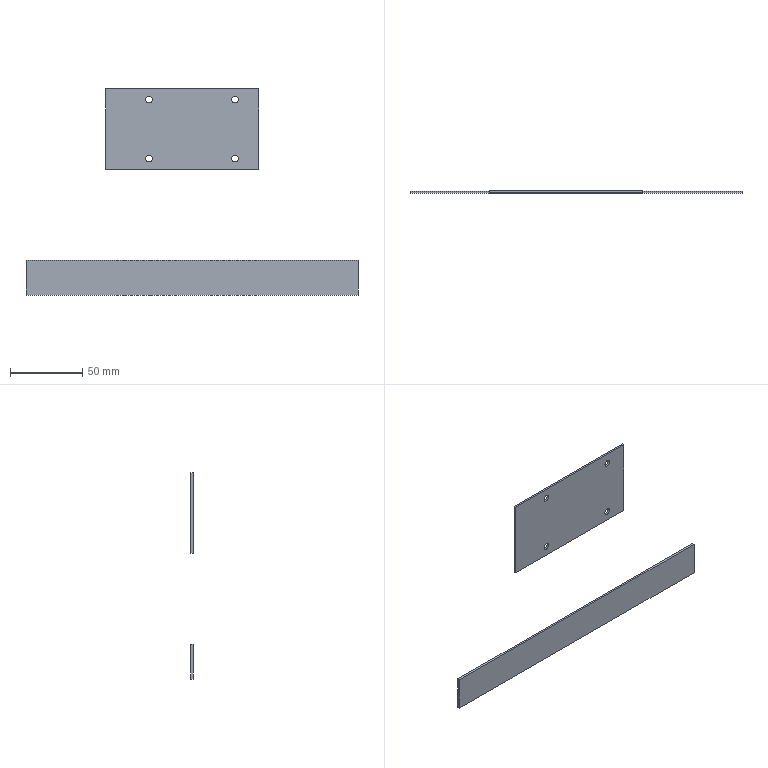Component | SolidWorks | CopperGasket-1 | 2 solids | 20 faces | box 230 x 1.5 x 142.89 mm | volume 17087 mm3 | plane 12 | cylinder 8 | commonest cylinder face diameters 4.542 x8
build123d program:
from build123d import *

# Parameters (mm, degrees)
SKETCH1_W           = 24.104
SKETCH1_H           = 230
BOSS_EXTRUDE1_DEPTH = 1.5
SKETCH3_W           = 55.775
SKETCH3_H           = 106
BOSS_EXTRUDE2_DEPTH = 1.5
SKETCH2_R           = 2.271
CUT_EXTRUDE1_DEPTH  = 210.219


with BuildPart() as part:
    # Sketch1 → Boss-Extrude1 (new body)
    with BuildSketch(Plane.XY):
        with Locations((102.948, -59.772)):
            Rectangle(SKETCH1_W, SKETCH1_H)
    extrude(amount=BOSS_EXTRUDE1_DEPTH)


with BuildPart() as body_2:
    # Sketch3 → Boss-Extrude2 (new body)
    with BuildSketch(Plane.XY.offset(1.5)):
        with Locations((0, -53)):
            Rectangle(SKETCH3_W, SKETCH3_H)
    extrude(amount=-BOSS_EXTRUDE2_DEPTH)

    # Sketch2 → Cut-Extrude1 (cut, through all)
    with BuildSketch(Plane.XY.offset(1.5)):
        with Locations((20.473, -29.973)):
            Circle(SKETCH2_R)
        with Locations((20.473, -89.571)):
            Circle(SKETCH2_R)
        with Locations((-20.473, -29.973)):
            Circle(SKETCH2_R)
        with Locations((-20.473, -89.571)):
            Circle(SKETCH2_R)
    extrude(amount=-CUT_EXTRUDE1_DEPTH, mode=Mode.SUBTRACT)


solid = Compound([part.part, body_2.part])

# Placed as in the assembly
solid = solid.moved(Location((-3, 95.24, 0), (-90, 0, 90)))
STEP:
#1=COLOUR_RGB('',0.7922,0.8196,0.9333);
#2=FILL_AREA_STYLE_COLOUR('',#1);
#3=FILL_AREA_STYLE('',(#2));
#4=SURFACE_STYLE_FILL_AREA(#3);
#5=SURFACE_SIDE_STYLE('',(#4));
#6=SURFACE_STYLE_USAGE(.BOTH.,#5);
#7=PRESENTATION_STYLE_ASSIGNMENT((#6));
#8=CARTESIAN_POINT('',(-2.292,3.75,-4.528));
#9=VERTEX_POINT('',#8);
#10=CARTESIAN_POINT('',(-2.292,3.75,-3.579));
#11=VERTEX_POINT('',#10);
#12=CARTESIAN_POINT('',(-2.292,3.75,-4.528));
#13=DIRECTION('',(0.,-0.,1.));
#14=VECTOR('',#13,39.37);
#15=LINE('',#12,#14);
#16=EDGE_CURVE('',#9,#11,#15,.T.);
#17=ORIENTED_EDGE('',*,*,#16,.T.);
#18=CARTESIAN_POINT('',(-2.292,3.809,-3.579));
#19=VERTEX_POINT('',#18);
#20=CARTESIAN_POINT('',(-2.292,3.809,-3.579));
#21=DIRECTION('',(0.,-1.,-0.));
#22=VECTOR('',#21,39.37);
#23=LINE('',#20,#22);
#24=EDGE_CURVE('',#19,#11,#23,.T.);
#25=ORIENTED_EDGE('',*,*,#24,.F.);
#26=CARTESIAN_POINT('',(-2.292,3.809,-4.528));
#27=VERTEX_POINT('',#26);
#28=CARTESIAN_POINT('',(-2.292,3.809,-4.528));
#29=DIRECTION('',(0.,-0.,1.));
#30=VECTOR('',#29,39.37);
#31=LINE('',#28,#30);
#32=EDGE_CURVE('',#27,#19,#31,.T.);
#33=ORIENTED_EDGE('',*,*,#32,.F.);
#34=CARTESIAN_POINT('',(-2.292,3.809,-4.528));
#35=DIRECTION('',(0.,-1.,-0.));
#36=VECTOR('',#35,39.37);
#37=LINE('',#34,#36);
#38=EDGE_CURVE('',#27,#9,#37,.T.);
#39=ORIENTED_EDGE('',*,*,#38,.T.);
#40=EDGE_LOOP('',(#17,#25,#33,#39));
#41=FACE_OUTER_BOUND('',#40,.T.);
#42=CARTESIAN_POINT('',(-2.292,3.809,-4.528));
#43=DIRECTION('',(1.,0.,-0.));
#44=DIRECTION('',(0.,-1.,-0.));
#45=AXIS2_PLACEMENT_3D('',#42,#43,#44);
#46=PLANE('',#45);
#47=ADVANCED_FACE('',(#41),#46,.F.);
#48=CARTESIAN_POINT('',(6.763,3.75,-3.579));
#49=VERTEX_POINT('',#48);
#50=CARTESIAN_POINT('',(-2.292,3.75,-3.579));
#51=DIRECTION('',(1.,-0.,0.));
#52=VECTOR('',#51,39.37);
#53=LINE('',#50,#52);
#54=EDGE_CURVE('',#11,#49,#53,.T.);
#55=ORIENTED_EDGE('',*,*,#54,.T.);
#56=CARTESIAN_POINT('',(6.763,3.809,-3.579));
#57=VERTEX_POINT('',#56);
#58=CARTESIAN_POINT('',(6.763,3.809,-3.579));
#59=DIRECTION('',(0.,-1.,-0.));
#60=VECTOR('',#59,39.37);
#61=LINE('',#58,#60);
#62=EDGE_CURVE('',#57,#49,#61,.T.);
#63=ORIENTED_EDGE('',*,*,#62,.F.);
#64=CARTESIAN_POINT('',(-2.292,3.809,-3.579));
#65=DIRECTION('',(1.,-0.,0.));
#66=VECTOR('',#65,39.37);
#67=LINE('',#64,#66);
#68=EDGE_CURVE('',#19,#57,#67,.T.);
#69=ORIENTED_EDGE('',*,*,#68,.F.);
#70=ORIENTED_EDGE('',*,*,#24,.T.);
#71=EDGE_LOOP('',(#55,#63,#69,#70));
#72=FACE_OUTER_BOUND('',#71,.T.);
#73=CARTESIAN_POINT('',(-2.292,3.809,-3.579));
#74=DIRECTION('',(0.,0.,-1.));
#75=DIRECTION('',(-1.,0.,-0.));
#76=AXIS2_PLACEMENT_3D('',#73,#74,#75);
#77=PLANE('',#76);
#78=ADVANCED_FACE('',(#72),#77,.F.);
#79=CARTESIAN_POINT('',(6.763,3.75,-4.528));
#80=VERTEX_POINT('',#79);
#81=CARTESIAN_POINT('',(6.763,3.75,-3.579));
#82=DIRECTION('',(0.,0.,-1.));
#83=VECTOR('',#82,39.37);
#84=LINE('',#81,#83);
#85=EDGE_CURVE('',#49,#80,#84,.T.);
#86=ORIENTED_EDGE('',*,*,#85,.T.);
#87=CARTESIAN_POINT('',(6.763,3.809,-4.528));
#88=VERTEX_POINT('',#87);
#89=CARTESIAN_POINT('',(6.763,3.809,-4.528));
#90=DIRECTION('',(0.,-1.,-0.));
#91=VECTOR('',#90,39.37);
#92=LINE('',#89,#91);
#93=EDGE_CURVE('',#88,#80,#92,.T.);
#94=ORIENTED_EDGE('',*,*,#93,.F.);
#95=CARTESIAN_POINT('',(6.763,3.809,-3.579));
#96=DIRECTION('',(0.,0.,-1.));
#97=VECTOR('',#96,39.37);
#98=LINE('',#95,#97);
#99=EDGE_CURVE('',#57,#88,#98,.T.);
#100=ORIENTED_EDGE('',*,*,#99,.F.);
#101=ORIENTED_EDGE('',*,*,#62,.T.);
#102=EDGE_LOOP('',(#86,#94,#100,#101));
#103=FACE_OUTER_BOUND('',#102,.T.);
#104=CARTESIAN_POINT('',(6.763,3.809,-3.579));
#105=DIRECTION('',(-1.,-0.,0.));
#106=DIRECTION('',(0.,1.,0.));
#107=AXIS2_PLACEMENT_3D('',#104,#105,#106);
#108=PLANE('',#107);
#109=ADVANCED_FACE('',(#103),#108,.F.);
#110=CARTESIAN_POINT('',(6.763,3.75,-4.528));
#111=DIRECTION('',(-1.,-0.,0.));
#112=VECTOR('',#111,39.37);
#113=LINE('',#110,#112);
#114=EDGE_CURVE('',#80,#9,#113,.T.);
#115=ORIENTED_EDGE('',*,*,#114,.T.);
#116=ORIENTED_EDGE('',*,*,#38,.F.);
#117=CARTESIAN_POINT('',(6.763,3.809,-4.528));
#118=DIRECTION('',(-1.,-0.,0.));
#119=VECTOR('',#118,39.37);
#120=LINE('',#117,#119);
#121=EDGE_CURVE('',#88,#27,#120,.T.);
#122=ORIENTED_EDGE('',*,*,#121,.F.);
#123=ORIENTED_EDGE('',*,*,#93,.T.);
#124=EDGE_LOOP('',(#115,#116,#122,#123));
#125=FACE_OUTER_BOUND('',#124,.T.);
#126=CARTESIAN_POINT('',(6.763,3.809,-4.528));
#127=DIRECTION('',(0.,-0.,1.));
#128=DIRECTION('',(1.,0.,-0.));
#129=AXIS2_PLACEMENT_3D('',#126,#127,#128);
#130=PLANE('',#129);
#131=ADVANCED_FACE('',(#125),#130,.F.);
#132=ORIENTED_EDGE('',*,*,#32,.T.);
#133=ORIENTED_EDGE('',*,*,#68,.T.);
#134=ORIENTED_EDGE('',*,*,#99,.T.);
#135=ORIENTED_EDGE('',*,*,#121,.T.);
#136=EDGE_LOOP('',(#132,#133,#134,#135));
#137=FACE_OUTER_BOUND('',#136,.T.);
#138=CARTESIAN_POINT('',(-0.1181,3.809,0.));
#139=DIRECTION('',(0.,1.,0.));
#140=DIRECTION('',(0.,0.,-1.));
#141=AXIS2_PLACEMENT_3D('',#138,#139,#140);
#142=PLANE('',#141);
#143=ADVANCED_FACE('',(#137),#142,.T.);
#144=ORIENTED_EDGE('',*,*,#16,.F.);
#145=ORIENTED_EDGE('',*,*,#114,.F.);
#146=ORIENTED_EDGE('',*,*,#85,.F.);
#147=ORIENTED_EDGE('',*,*,#54,.F.);
#148=EDGE_LOOP('',(#144,#145,#146,#147));
#149=FACE_OUTER_BOUND('',#148,.T.);
#150=CARTESIAN_POINT('',(-0.1181,3.75,0.));
#151=DIRECTION('',(0.,1.,0.));
#152=DIRECTION('',(0.,0.,-1.));
#153=AXIS2_PLACEMENT_3D('',#150,#151,#152);
#154=PLANE('',#153);
#155=ADVANCED_FACE('',(#149),#154,.F.);
#156=CLOSED_SHELL('',(#47,#78,#109,#131,#143,#155));
#157=MANIFOLD_SOLID_BREP('',#156);
#158=STYLED_ITEM('',(#7),#157);
#159=PRESENTATION_LAYER_ASSIGNMENT('','',(#158));
#160=(LENGTH_UNIT()NAMED_UNIT(*)SI_UNIT($,.METRE.));
#161=LENGTH_MEASURE_WITH_UNIT(LENGTH_MEASURE(0.0254),#160);
#162=DIMENSIONAL_EXPONENTS(1.,0.,0.,0.,0.,0.,0.);
#163=(CONVERSION_BASED_UNIT('',#161)LENGTH_UNIT()NAMED_UNIT(#162));
#164=UNCERTAINTY_MEASURE_WITH_UNIT(LENGTH_MEASURE(0.00001),#163,'','');
#165=(NAMED_UNIT(*)PLANE_ANGLE_UNIT()SI_UNIT($,.RADIAN.));
#166=(NAMED_UNIT(*)SI_UNIT($,.STERADIAN.)SOLID_ANGLE_UNIT());
#167=(GEOMETRIC_REPRESENTATION_CONTEXT(3)GLOBAL_UNCERTAINTY_ASSIGNED_CONTEXT((#164))GLOBAL_UNIT_ASSIGNED_CONTEXT((#163,#165,#166))REPRESENTATION_CONTEXT('',''));
#168=MECHANICAL_DESIGN_GEOMETRIC_PRESENTATION_REPRESENTATION('',(#158),#167);
#169=COLOUR_RGB('',0.7922,0.8196,0.9333);
#170=FILL_AREA_STYLE_COLOUR('',#169);
#171=FILL_AREA_STYLE('',(#170));
#172=SURFACE_STYLE_FILL_AREA(#171);
#173=SURFACE_SIDE_STYLE('',(#172));
#174=SURFACE_STYLE_USAGE(.BOTH.,#173);
#175=PRESENTATION_STYLE_ASSIGNMENT((#174));
#176=CARTESIAN_POINT('',(3.408,3.75,-0.7166));
#177=VERTEX_POINT('',#176);
#178=CARTESIAN_POINT('',(3.408,3.75,-0.8954));
#179=VERTEX_POINT('',#178);
#180=CARTESIAN_POINT('',(3.408,3.75,-0.806));
#181=DIRECTION('',(0.,1.,0.));
#182=DIRECTION('',(0.,0.,-1.));
#183=AXIS2_PLACEMENT_3D('',#180,#181,#182);
#184=CIRCLE('',#183,0.08941);
#185=EDGE_CURVE('',#177,#179,#184,.T.);
#186=ORIENTED_EDGE('',*,*,#185,.F.);
#187=CARTESIAN_POINT('',(3.408,3.809,-0.7166));
#188=VERTEX_POINT('',#187);
#189=CARTESIAN_POINT('',(3.408,3.75,-0.7166));
#190=DIRECTION('',(0.,1.,0.));
#191=VECTOR('',#190,39.37);
#192=LINE('',#189,#191);
#193=EDGE_CURVE('',#177,#188,#192,.T.);
#194=ORIENTED_EDGE('',*,*,#193,.T.);
#195=CARTESIAN_POINT('',(3.408,3.809,-0.8954));
#196=VERTEX_POINT('',#195);
#197=CARTESIAN_POINT('',(3.408,3.809,-0.806));
#198=DIRECTION('',(0.,1.,0.));
#199=DIRECTION('',(0.,0.,-1.));
#200=AXIS2_PLACEMENT_3D('',#197,#198,#199);
#201=CIRCLE('',#200,0.08941);
#202=EDGE_CURVE('',#188,#196,#201,.T.);
#203=ORIENTED_EDGE('',*,*,#202,.T.);
#204=CARTESIAN_POINT('',(3.408,3.75,-0.8954));
#205=DIRECTION('',(0.,1.,0.));
#206=VECTOR('',#205,39.37);
#207=LINE('',#204,#206);
#208=EDGE_CURVE('',#179,#196,#207,.T.);
#209=ORIENTED_EDGE('',*,*,#208,.F.);
#210=EDGE_LOOP('',(#186,#194,#203,#209));
#211=FACE_OUTER_BOUND('',#210,.T.);
#212=CARTESIAN_POINT('',(3.408,3.75,-0.806));
#213=DIRECTION('',(0.,1.,0.));
#214=DIRECTION('',(0.,0.,-1.));
#215=AXIS2_PLACEMENT_3D('',#212,#213,#214);
#216=CYLINDRICAL_SURFACE('',#215,0.08941);
#217=ADVANCED_FACE('',(#211),#216,.F.);
#218=CARTESIAN_POINT('',(1.062,3.75,0.8954));
#219=VERTEX_POINT('',#218);
#220=CARTESIAN_POINT('',(1.062,3.75,0.7166));
#221=VERTEX_POINT('',#220);
#222=CARTESIAN_POINT('',(1.062,3.75,0.806));
#223=DIRECTION('',(0.,1.,0.));
#224=DIRECTION('',(0.,0.,-1.));
#225=AXIS2_PLACEMENT_3D('',#222,#223,#224);
#226=CIRCLE('',#225,0.08941);
#227=EDGE_CURVE('',#219,#221,#226,.T.);
#228=ORIENTED_EDGE('',*,*,#227,.F.);
#229=CARTESIAN_POINT('',(1.062,3.809,0.8954));
#230=VERTEX_POINT('',#229);
#231=CARTESIAN_POINT('',(1.062,3.75,0.8954));
#232=DIRECTION('',(0.,1.,0.));
#233=VECTOR('',#232,39.37);
#234=LINE('',#231,#233);
#235=EDGE_CURVE('',#219,#230,#234,.T.);
#236=ORIENTED_EDGE('',*,*,#235,.T.);
#237=CARTESIAN_POINT('',(1.062,3.809,0.7166));
#238=VERTEX_POINT('',#237);
#239=CARTESIAN_POINT('',(1.062,3.809,0.806));
#240=DIRECTION('',(0.,1.,0.));
#241=DIRECTION('',(0.,0.,-1.));
#242=AXIS2_PLACEMENT_3D('',#239,#240,#241);
#243=CIRCLE('',#242,0.08941);
#244=EDGE_CURVE('',#230,#238,#243,.T.);
#245=ORIENTED_EDGE('',*,*,#244,.T.);
#246=CARTESIAN_POINT('',(1.062,3.75,0.7166));
#247=DIRECTION('',(0.,1.,0.));
#248=VECTOR('',#247,39.37);
#249=LINE('',#246,#248);
#250=EDGE_CURVE('',#221,#238,#249,.T.);
#251=ORIENTED_EDGE('',*,*,#250,.F.);
#252=EDGE_LOOP('',(#228,#236,#245,#251));
#253=FACE_OUTER_BOUND('',#252,.T.);
#254=CARTESIAN_POINT('',(1.062,3.75,0.806));
#255=DIRECTION('',(0.,1.,0.));
#256=DIRECTION('',(0.,0.,-1.));
#257=AXIS2_PLACEMENT_3D('',#254,#255,#256);
#258=CYLINDRICAL_SURFACE('',#257,0.08941);
#259=ADVANCED_FACE('',(#253),#258,.F.);
#260=CARTESIAN_POINT('',(3.408,3.75,0.8954));
#261=VERTEX_POINT('',#260);
#262=CARTESIAN_POINT('',(3.408,3.75,0.7166));
#263=VERTEX_POINT('',#262);
#264=CARTESIAN_POINT('',(3.408,3.75,0.806));
#265=DIRECTION('',(0.,1.,0.));
#266=DIRECTION('',(0.,0.,-1.));
#267=AXIS2_PLACEMENT_3D('',#264,#265,#266);
#268=CIRCLE('',#267,0.08941);
#269=EDGE_CURVE('',#261,#263,#268,.T.);
#270=ORIENTED_EDGE('',*,*,#269,.F.);
#271=CARTESIAN_POINT('',(3.408,3.809,0.8954));
#272=VERTEX_POINT('',#271);
#273=CARTESIAN_POINT('',(3.408,3.75,0.8954));
#274=DIRECTION('',(0.,1.,0.));
#275=VECTOR('',#274,39.37);
#276=LINE('',#273,#275);
#277=EDGE_CURVE('',#261,#272,#276,.T.);
#278=ORIENTED_EDGE('',*,*,#277,.T.);
#279=CARTESIAN_POINT('',(3.408,3.809,0.7166));
#280=VERTEX_POINT('',#279);
#281=CARTESIAN_POINT('',(3.408,3.809,0.806));
#282=DIRECTION('',(0.,1.,0.));
#283=DIRECTION('',(0.,0.,-1.));
#284=AXIS2_PLACEMENT_3D('',#281,#282,#283);
#285=CIRCLE('',#284,0.08941);
#286=EDGE_CURVE('',#272,#280,#285,.T.);
#287=ORIENTED_EDGE('',*,*,#286,.T.);
#288=CARTESIAN_POINT('',(3.408,3.75,0.7166));
#289=DIRECTION('',(0.,1.,0.));
#290=VECTOR('',#289,39.37);
#291=LINE('',#288,#290);
#292=EDGE_CURVE('',#263,#280,#291,.T.);
#293=ORIENTED_EDGE('',*,*,#292,.F.);
#294=EDGE_LOOP('',(#270,#278,#287,#293));
#295=FACE_OUTER_BOUND('',#294,.T.);
#296=CARTESIAN_POINT('',(3.408,3.75,0.806));
#297=DIRECTION('',(0.,1.,0.));
#298=DIRECTION('',(0.,0.,-1.));
#299=AXIS2_PLACEMENT_3D('',#296,#297,#298);
#300=CYLINDRICAL_SURFACE('',#299,0.08941);
#301=ADVANCED_FACE('',(#295),#300,.F.);
#302=CARTESIAN_POINT('',(1.062,3.75,-0.7166));
#303=VERTEX_POINT('',#302);
#304=CARTESIAN_POINT('',(1.062,3.75,-0.8954));
#305=VERTEX_POINT('',#304);
#306=CARTESIAN_POINT('',(1.062,3.75,-0.806));
#307=DIRECTION('',(0.,1.,0.));
#308=DIRECTION('',(0.,0.,-1.));
#309=AXIS2_PLACEMENT_3D('',#306,#307,#308);
#310=CIRCLE('',#309,0.08941);
#311=EDGE_CURVE('',#303,#305,#310,.T.);
#312=ORIENTED_EDGE('',*,*,#311,.F.);
#313=CARTESIAN_POINT('',(1.062,3.809,-0.7166));
#314=VERTEX_POINT('',#313);
#315=CARTESIAN_POINT('',(1.062,3.75,-0.7166));
#316=DIRECTION('',(0.,1.,0.));
#317=VECTOR('',#316,39.37);
#318=LINE('',#315,#317);
#319=EDGE_CURVE('',#303,#314,#318,.T.);
#320=ORIENTED_EDGE('',*,*,#319,.T.);
#321=CARTESIAN_POINT('',(1.062,3.809,-0.8954));
#322=VERTEX_POINT('',#321);
#323=CARTESIAN_POINT('',(1.062,3.809,-0.806));
#324=DIRECTION('',(0.,1.,0.));
#325=DIRECTION('',(0.,0.,-1.));
#326=AXIS2_PLACEMENT_3D('',#323,#324,#325);
#327=CIRCLE('',#326,0.08941);
#328=EDGE_CURVE('',#314,#322,#327,.T.);
#329=ORIENTED_EDGE('',*,*,#328,.T.);
#330=CARTESIAN_POINT('',(1.062,3.75,-0.8954));
#331=DIRECTION('',(0.,1.,0.));
#332=VECTOR('',#331,39.37);
#333=LINE('',#330,#332);
#334=EDGE_CURVE('',#305,#322,#333,.T.);
#335=ORIENTED_EDGE('',*,*,#334,.F.);
#336=EDGE_LOOP('',(#312,#320,#329,#335));
#337=FACE_OUTER_BOUND('',#336,.T.);
#338=CARTESIAN_POINT('',(1.062,3.75,-0.806));
#339=DIRECTION('',(0.,1.,0.));
#340=DIRECTION('',(0.,0.,-1.));
#341=AXIS2_PLACEMENT_3D('',#338,#339,#340);
#342=CYLINDRICAL_SURFACE('',#341,0.08941);
#343=ADVANCED_FACE('',(#337),#342,.F.);
#344=CARTESIAN_POINT('',(4.055,3.809,1.098));
#345=VERTEX_POINT('',#344);
#346=CARTESIAN_POINT('',(-0.1181,3.809,1.098));
#347=VERTEX_POINT('',#346);
#348=CARTESIAN_POINT('',(-0.1181,3.809,1.098));
#349=DIRECTION('',(-1.,0.,0.));
#350=VECTOR('',#349,39.37);
#351=LINE('',#348,#350);
#352=EDGE_CURVE('',#345,#347,#351,.T.);
#353=ORIENTED_EDGE('',*,*,#352,.T.);
#354=CARTESIAN_POINT('',(-0.1181,3.75,1.098));
#355=VERTEX_POINT('',#354);
#356=CARTESIAN_POINT('',(-0.1181,3.75,1.098));
#357=DIRECTION('',(0.,1.,0.));
#358=VECTOR('',#357,39.37);
#359=LINE('',#356,#358);
#360=EDGE_CURVE('',#355,#347,#359,.T.);
#361=ORIENTED_EDGE('',*,*,#360,.F.);
#362=CARTESIAN_POINT('',(4.055,3.75,1.098));
#363=VERTEX_POINT('',#362);
#364=CARTESIAN_POINT('',(-0.1181,3.75,1.098));
#365=DIRECTION('',(-1.,0.,0.));
#366=VECTOR('',#365,39.37);
#367=LINE('',#364,#366);
#368=EDGE_CURVE('',#363,#355,#367,.T.);
#369=ORIENTED_EDGE('',*,*,#368,.F.);
#370=CARTESIAN_POINT('',(4.055,3.75,1.098));
#371=DIRECTION('',(0.,1.,0.));
#372=VECTOR('',#371,39.37);
#373=LINE('',#370,#372);
#374=EDGE_CURVE('',#363,#345,#373,.T.);
#375=ORIENTED_EDGE('',*,*,#374,.T.);
#376=EDGE_LOOP('',(#353,#361,#369,#375));
#377=FACE_OUTER_BOUND('',#376,.T.);
#378=CARTESIAN_POINT('',(-0.1181,3.75,1.098));
#379=DIRECTION('',(0.,0.,-1.));
#380=DIRECTION('',(0.,-1.,-0.));
#381=AXIS2_PLACEMENT_3D('',#378,#379,#380);
#382=PLANE('',#381);
#383=ADVANCED_FACE('',(#377),#382,.F.);
#384=CARTESIAN_POINT('',(-0.1181,3.809,-1.098));
#385=VERTEX_POINT('',#384);
#386=CARTESIAN_POINT('',(-0.1181,3.809,0.));
#387=DIRECTION('',(0.,-0.,1.));
#388=VECTOR('',#387,39.37);
#389=LINE('',#386,#388);
#390=EDGE_CURVE('',#385,#347,#389,.T.);
#391=ORIENTED_EDGE('',*,*,#390,.F.);
#392=CARTESIAN_POINT('',(-0.1181,3.75,-1.098));
#393=VERTEX_POINT('',#392);
#394=CARTESIAN_POINT('',(-0.1181,3.75,-1.098));
#395=DIRECTION('',(0.,1.,0.));
#396=VECTOR('',#395,39.37);
#397=LINE('',#394,#396);
#398=EDGE_CURVE('',#393,#385,#397,.T.);
#399=ORIENTED_EDGE('',*,*,#398,.F.);
#400=CARTESIAN_POINT('',(-0.1181,3.75,0.));
#401=DIRECTION('',(0.,-0.,1.));
#402=VECTOR('',#401,39.37);
#403=LINE('',#400,#402);
#404=EDGE_CURVE('',#393,#355,#403,.T.);
#405=ORIENTED_EDGE('',*,*,#404,.T.);
#406=ORIENTED_EDGE('',*,*,#360,.T.);
#407=EDGE_LOOP('',(#391,#399,#405,#406));
#408=FACE_OUTER_BOUND('',#407,.T.);
#409=CARTESIAN_POINT('',(-0.1181,3.75,0.));
#410=DIRECTION('',(-1.,-0.,0.));
#411=DIRECTION('',(0.,1.,0.));
#412=AXIS2_PLACEMENT_3D('',#409,#410,#411);
#413=PLANE('',#412);
#414=ADVANCED_FACE('',(#408),#413,.T.);
#415=CARTESIAN_POINT('',(4.055,3.809,-1.098));
#416=VERTEX_POINT('',#415);
#417=CARTESIAN_POINT('',(-0.1181,3.809,-1.098));
#418=DIRECTION('',(-1.,0.,0.));
#419=VECTOR('',#418,39.37);
#420=LINE('',#417,#419);
#421=EDGE_CURVE('',#416,#385,#420,.T.);
#422=ORIENTED_EDGE('',*,*,#421,.F.);
#423=CARTESIAN_POINT('',(4.055,3.75,-1.098));
#424=VERTEX_POINT('',#423);
#425=CARTESIAN_POINT('',(4.055,3.75,-1.098));
#426=DIRECTION('',(0.,1.,0.));
#427=VECTOR('',#426,39.37);
#428=LINE('',#425,#427);
#429=EDGE_CURVE('',#424,#416,#428,.T.);
#430=ORIENTED_EDGE('',*,*,#429,.F.);
#431=CARTESIAN_POINT('',(-0.1181,3.75,-1.098));
#432=DIRECTION('',(-1.,0.,0.));
#433=VECTOR('',#432,39.37);
#434=LINE('',#431,#433);
#435=EDGE_CURVE('',#424,#393,#434,.T.);
#436=ORIENTED_EDGE('',*,*,#435,.T.);
#437=ORIENTED_EDGE('',*,*,#398,.T.);
#438=EDGE_LOOP('',(#422,#430,#436,#437));
#439=FACE_OUTER_BOUND('',#438,.T.);
#440=CARTESIAN_POINT('',(-0.1181,3.75,-1.098));
#441=DIRECTION('',(0.,0.,-1.));
#442=DIRECTION('',(0.,-1.,-0.));
#443=AXIS2_PLACEMENT_3D('',#440,#441,#442);
#444=PLANE('',#443);
#445=ADVANCED_FACE('',(#439),#444,.T.);
#446=CARTESIAN_POINT('',(4.055,3.809,0.));
#447=DIRECTION('',(0.,-0.,1.));
#448=VECTOR('',#447,39.37);
#449=LINE('',#446,#448);
#450=EDGE_CURVE('',#416,#345,#449,.T.);
#451=ORIENTED_EDGE('',*,*,#450,.T.);
#452=ORIENTED_EDGE('',*,*,#374,.F.);
#453=CARTESIAN_POINT('',(4.055,3.75,0.));
#454=DIRECTION('',(0.,-0.,1.));
#455=VECTOR('',#454,39.37);
#456=LINE('',#453,#455);
#457=EDGE_CURVE('',#424,#363,#456,.T.);
#458=ORIENTED_EDGE('',*,*,#457,.F.);
#459=ORIENTED_EDGE('',*,*,#429,.T.);
#460=EDGE_LOOP('',(#451,#452,#458,#459));
#461=FACE_OUTER_BOUND('',#460,.T.);
#462=CARTESIAN_POINT('',(4.055,3.75,0.));
#463=DIRECTION('',(-1.,-0.,0.));
#464=DIRECTION('',(0.,1.,0.));
#465=AXIS2_PLACEMENT_3D('',#462,#463,#464);
#466=PLANE('',#465);
#467=ADVANCED_FACE('',(#461),#466,.F.);
#468=CARTESIAN_POINT('',(3.408,3.75,-0.806));
#469=DIRECTION('',(0.,1.,0.));
#470=DIRECTION('',(0.,0.,-1.));
#471=AXIS2_PLACEMENT_3D('',#468,#469,#470);
#472=CIRCLE('',#471,0.08941);
#473=EDGE_CURVE('',#179,#177,#472,.T.);
#474=ORIENTED_EDGE('',*,*,#473,.T.);
#475=ORIENTED_EDGE('',*,*,#185,.T.);
#476=EDGE_LOOP('',(#474,#475));
#477=FACE_BOUND('',#476,.T.);
#478=CARTESIAN_POINT('',(1.062,3.75,0.806));
#479=DIRECTION('',(0.,1.,0.));
#480=DIRECTION('',(0.,0.,-1.));
#481=AXIS2_PLACEMENT_3D('',#478,#479,#480);
#482=CIRCLE('',#481,0.08941);
#483=EDGE_CURVE('',#221,#219,#482,.T.);
#484=ORIENTED_EDGE('',*,*,#483,.T.);
#485=ORIENTED_EDGE('',*,*,#227,.T.);
#486=EDGE_LOOP('',(#484,#485));
#487=FACE_BOUND('',#486,.T.);
#488=CARTESIAN_POINT('',(3.408,3.75,0.806));
#489=DIRECTION('',(0.,1.,0.));
#490=DIRECTION('',(0.,0.,-1.));
#491=AXIS2_PLACEMENT_3D('',#488,#489,#490);
#492=CIRCLE('',#491,0.08941);
#493=EDGE_CURVE('',#263,#261,#492,.T.);
#494=ORIENTED_EDGE('',*,*,#493,.T.);
#495=ORIENTED_EDGE('',*,*,#269,.T.);
#496=EDGE_LOOP('',(#494,#495));
#497=FACE_BOUND('',#496,.T.);
#498=CARTESIAN_POINT('',(1.062,3.75,-0.806));
#499=DIRECTION('',(0.,1.,0.));
#500=DIRECTION('',(0.,0.,-1.));
#501=AXIS2_PLACEMENT_3D('',#498,#499,#500);
#502=CIRCLE('',#501,0.08941);
#503=EDGE_CURVE('',#305,#303,#502,.T.);
#504=ORIENTED_EDGE('',*,*,#503,.T.);
#505=ORIENTED_EDGE('',*,*,#311,.T.);
#506=EDGE_LOOP('',(#504,#505));
#507=FACE_BOUND('',#506,.T.);
#508=ORIENTED_EDGE('',*,*,#368,.T.);
#509=ORIENTED_EDGE('',*,*,#404,.F.);
#510=ORIENTED_EDGE('',*,*,#435,.F.);
#511=ORIENTED_EDGE('',*,*,#457,.T.);
#512=EDGE_LOOP('',(#508,#509,#510,#511));
#513=FACE_OUTER_BOUND('',#512,.T.);
#514=CARTESIAN_POINT('',(-0.1181,3.75,0.));
#515=DIRECTION('',(0.,1.,0.));
#516=DIRECTION('',(0.,0.,-1.));
#517=AXIS2_PLACEMENT_3D('',#514,#515,#516);
#518=PLANE('',#517);
#519=ADVANCED_FACE('',(#477,#487,#497,#507,#513),#518,.F.);
#520=CARTESIAN_POINT('',(3.408,3.809,-0.806));
#521=DIRECTION('',(0.,1.,0.));
#522=DIRECTION('',(0.,0.,-1.));
#523=AXIS2_PLACEMENT_3D('',#520,#521,#522);
#524=CIRCLE('',#523,0.08941);
#525=EDGE_CURVE('',#196,#188,#524,.T.);
#526=ORIENTED_EDGE('',*,*,#525,.F.);
#527=ORIENTED_EDGE('',*,*,#202,.F.);
#528=EDGE_LOOP('',(#526,#527));
#529=FACE_BOUND('',#528,.T.);
#530=CARTESIAN_POINT('',(1.062,3.809,0.806));
#531=DIRECTION('',(0.,1.,0.));
#532=DIRECTION('',(0.,0.,-1.));
#533=AXIS2_PLACEMENT_3D('',#530,#531,#532);
#534=CIRCLE('',#533,0.08941);
#535=EDGE_CURVE('',#238,#230,#534,.T.);
#536=ORIENTED_EDGE('',*,*,#535,.F.);
#537=ORIENTED_EDGE('',*,*,#244,.F.);
#538=EDGE_LOOP('',(#536,#537));
#539=FACE_BOUND('',#538,.T.);
#540=CARTESIAN_POINT('',(3.408,3.809,0.806));
#541=DIRECTION('',(0.,1.,0.));
#542=DIRECTION('',(0.,0.,-1.));
#543=AXIS2_PLACEMENT_3D('',#540,#541,#542);
#544=CIRCLE('',#543,0.08941);
#545=EDGE_CURVE('',#280,#272,#544,.T.);
#546=ORIENTED_EDGE('',*,*,#545,.F.);
#547=ORIENTED_EDGE('',*,*,#286,.F.);
#548=EDGE_LOOP('',(#546,#547));
#549=FACE_BOUND('',#548,.T.);
#550=CARTESIAN_POINT('',(1.062,3.809,-0.806));
#551=DIRECTION('',(0.,1.,0.));
#552=DIRECTION('',(0.,0.,-1.));
#553=AXIS2_PLACEMENT_3D('',#550,#551,#552);
#554=CIRCLE('',#553,0.08941);
#555=EDGE_CURVE('',#322,#314,#554,.T.);
#556=ORIENTED_EDGE('',*,*,#555,.F.);
#557=ORIENTED_EDGE('',*,*,#328,.F.);
#558=EDGE_LOOP('',(#556,#557));
#559=FACE_BOUND('',#558,.T.);
#560=ORIENTED_EDGE('',*,*,#352,.F.);
#561=ORIENTED_EDGE('',*,*,#450,.F.);
#562=ORIENTED_EDGE('',*,*,#421,.T.);
#563=ORIENTED_EDGE('',*,*,#390,.T.);
#564=EDGE_LOOP('',(#560,#561,#562,#563));
#565=FACE_OUTER_BOUND('',#564,.T.);
#566=CARTESIAN_POINT('',(-0.1181,3.809,0.));
#567=DIRECTION('',(0.,1.,0.));
#568=DIRECTION('',(0.,0.,-1.));
#569=AXIS2_PLACEMENT_3D('',#566,#567,#568);
#570=PLANE('',#569);
#571=ADVANCED_FACE('',(#529,#539,#549,#559,#565),#570,.T.);
#572=ORIENTED_EDGE('',*,*,#319,.F.);
#573=ORIENTED_EDGE('',*,*,#503,.F.);
#574=ORIENTED_EDGE('',*,*,#334,.T.);
#575=ORIENTED_EDGE('',*,*,#555,.T.);
#576=EDGE_LOOP('',(#572,#573,#574,#575));
#577=FACE_OUTER_BOUND('',#576,.T.);
#578=CARTESIAN_POINT('',(1.062,3.75,-0.806));
#579=DIRECTION('',(0.,1.,0.));
#580=DIRECTION('',(0.,0.,-1.));
#581=AXIS2_PLACEMENT_3D('',#578,#579,#580);
#582=CYLINDRICAL_SURFACE('',#581,0.08941);
#583=ADVANCED_FACE('',(#577),#582,.F.);
#584=ORIENTED_EDGE('',*,*,#277,.F.);
#585=ORIENTED_EDGE('',*,*,#493,.F.);
#586=ORIENTED_EDGE('',*,*,#292,.T.);
#587=ORIENTED_EDGE('',*,*,#545,.T.);
#588=EDGE_LOOP('',(#584,#585,#586,#587));
#589=FACE_OUTER_BOUND('',#588,.T.);
#590=CARTESIAN_POINT('',(3.408,3.75,0.806));
#591=DIRECTION('',(0.,1.,0.));
#592=DIRECTION('',(0.,0.,-1.));
#593=AXIS2_PLACEMENT_3D('',#590,#591,#592);
#594=CYLINDRICAL_SURFACE('',#593,0.08941);
#595=ADVANCED_FACE('',(#589),#594,.F.);
#596=ORIENTED_EDGE('',*,*,#235,.F.);
#597=ORIENTED_EDGE('',*,*,#483,.F.);
#598=ORIENTED_EDGE('',*,*,#250,.T.);
#599=ORIENTED_EDGE('',*,*,#535,.T.);
#600=EDGE_LOOP('',(#596,#597,#598,#599));
#601=FACE_OUTER_BOUND('',#600,.T.);
#602=CARTESIAN_POINT('',(1.062,3.75,0.806));
#603=DIRECTION('',(0.,1.,0.));
#604=DIRECTION('',(0.,0.,-1.));
#605=AXIS2_PLACEMENT_3D('',#602,#603,#604);
#606=CYLINDRICAL_SURFACE('',#605,0.08941);
#607=ADVANCED_FACE('',(#601),#606,.F.);
#608=ORIENTED_EDGE('',*,*,#193,.F.);
#609=ORIENTED_EDGE('',*,*,#473,.F.);
#610=ORIENTED_EDGE('',*,*,#208,.T.);
#611=ORIENTED_EDGE('',*,*,#525,.T.);
#612=EDGE_LOOP('',(#608,#609,#610,#611));
#613=FACE_OUTER_BOUND('',#612,.T.);
#614=CARTESIAN_POINT('',(3.408,3.75,-0.806));
#615=DIRECTION('',(0.,1.,0.));
#616=DIRECTION('',(0.,0.,-1.));
#617=AXIS2_PLACEMENT_3D('',#614,#615,#616);
#618=CYLINDRICAL_SURFACE('',#617,0.08941);
#619=ADVANCED_FACE('',(#613),#618,.F.);
#620=CLOSED_SHELL('',(#217,#259,#301,#343,#383,#414,#445,#467,#519,#571,#583,#595,#607,#619));
#621=MANIFOLD_SOLID_BREP('',#620);
#622=STYLED_ITEM('',(#175),#621);
#623=(LENGTH_UNIT()NAMED_UNIT(*)SI_UNIT($,.METRE.));
#624=LENGTH_MEASURE_WITH_UNIT(LENGTH_MEASURE(0.0254),#623);
#625=DIMENSIONAL_EXPONENTS(1.,0.,0.,0.,0.,0.,0.);
#626=(CONVERSION_BASED_UNIT('',#624)LENGTH_UNIT()NAMED_UNIT(#625));
#627=UNCERTAINTY_MEASURE_WITH_UNIT(LENGTH_MEASURE(0.00001),#626,'','');
#628=(NAMED_UNIT(*)PLANE_ANGLE_UNIT()SI_UNIT($,.RADIAN.));
#629=(NAMED_UNIT(*)SI_UNIT($,.STERADIAN.)SOLID_ANGLE_UNIT());
#630=(GEOMETRIC_REPRESENTATION_CONTEXT(3)GLOBAL_UNCERTAINTY_ASSIGNED_CONTEXT((#627))GLOBAL_UNIT_ASSIGNED_CONTEXT((#626,#628,#629))REPRESENTATION_CONTEXT('',''));
#631=MECHANICAL_DESIGN_GEOMETRIC_PRESENTATION_REPRESENTATION('',(#622),#630);
#632=PRESENTATION_LAYER_ASSIGNMENT('','',(#622));
#633=CARTESIAN_POINT('',(0.,0.,0.));
#634=DIRECTION('',(0.,0.,1.));
#635=DIRECTION('',(1.,0.,0.));
#636=AXIS2_PLACEMENT_3D('',#633,#634,#635);
#637=(LENGTH_UNIT()NAMED_UNIT(*)SI_UNIT($,.METRE.));
#638=LENGTH_MEASURE_WITH_UNIT(LENGTH_MEASURE(0.0254),#637);
#639=DIMENSIONAL_EXPONENTS(1.,0.,0.,0.,0.,0.,0.);
#640=(CONVERSION_BASED_UNIT('',#638)LENGTH_UNIT()NAMED_UNIT(#639));
#641=UNCERTAINTY_MEASURE_WITH_UNIT(LENGTH_MEASURE(0.00001),#640,'','');
#642=(NAMED_UNIT(*)PLANE_ANGLE_UNIT()SI_UNIT($,.RADIAN.));
#643=(NAMED_UNIT(*)SI_UNIT($,.STERADIAN.)SOLID_ANGLE_UNIT());
#644=(GEOMETRIC_REPRESENTATION_CONTEXT(3)GLOBAL_UNCERTAINTY_ASSIGNED_CONTEXT((#641))GLOBAL_UNIT_ASSIGNED_CONTEXT((#640,#642,#643))REPRESENTATION_CONTEXT('',''));
#645=ADVANCED_BREP_SHAPE_REPRESENTATION('',(#621,#157,#636),#644);